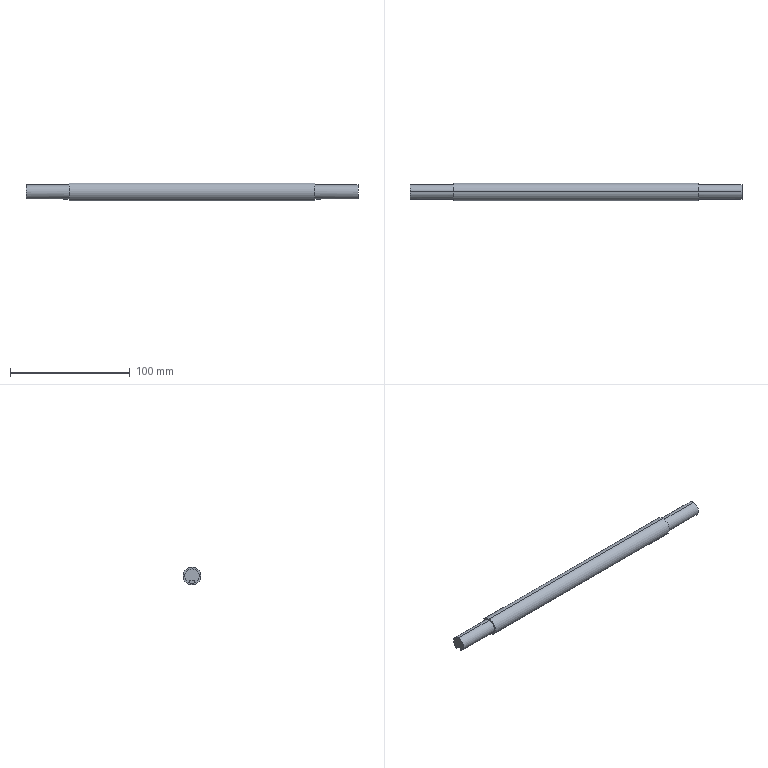Component | SolidWorks | ReducerCoupling-1 | 1 solid | 18 faces | box 277 x 15 x 15 mm | volume 43778 mm3 | plane 12 | cylinder 6 | commonest cylinder face diameters 12 x4 15 x2
build123d program:
from build123d import *

# Parameters (mm, degrees)
SKETCH2_W      = 4
SKETCH2_H      = 3.974
EXTRUDE1_DEPTH = 31
SKETCH3_W      = 4
SKETCH3_H      = 4.547
EXTRUDE2_DEPTH = 31


with BuildPart() as part:
    # Sketch1 → Revolve1 (revolve)
    with BuildSketch(Plane.XY, mode=Mode.PRIVATE) as revolve1_sk:
        Polygon((0, 106.041), (6, 106.041), (6, 70.041), (7.5, 70.041), (7.5, -134.959), (6, -134.959), (6, -170.959), (0, -170.959), align=None)
    revolve(revolve1_sk.sketch.rotate(Axis((0, 0, 0), (0, 1, 0)), 90), axis=Axis((0, 0, 0), (0, 1, 0)))

    # Sketch2 → Extrude1 (cut)
    with BuildSketch(Plane(origin=(0, 106.041, 0), x_dir=(1, 0, 0), z_dir=(0, 1, 0))):
        with Locations((0, 5.487)):
            Rectangle(SKETCH2_W, SKETCH2_H)
    extrude(amount=-EXTRUDE1_DEPTH, mode=Mode.SUBTRACT)

    # Sketch3 → Extrude2 (cut)
    with BuildSketch(Plane.XZ.offset(170.959)):
        with Locations((0, -5.774)):
            Rectangle(SKETCH3_W, SKETCH3_H)
    extrude(amount=-EXTRUDE2_DEPTH, mode=Mode.SUBTRACT)


solid = part.part

# Placed as in the assembly
solid = solid.moved(Location((52.758, 175.983, 58.736), (0, 0, 90)))
STEP:
#1=COLOUR_RGB('',0.7922,0.8196,0.9333);
#2=FILL_AREA_STYLE_COLOUR('',#1);
#3=FILL_AREA_STYLE('',(#2));
#4=SURFACE_STYLE_FILL_AREA(#3);
#5=SURFACE_SIDE_STYLE('',(#4));
#6=SURFACE_STYLE_USAGE(.BOTH.,#5);
#7=PRESENTATION_STYLE_ASSIGNMENT((#6));
#8=CARTESIAN_POINT('',(7.39,6.928,2.076));
#9=VERTEX_POINT('',#8);
#10=CARTESIAN_POINT('',(7.39,6.928,2.549));
#11=VERTEX_POINT('',#10);
#12=CARTESIAN_POINT('',(7.39,6.928,2.312));
#13=DIRECTION('',(1.,0.,0.));
#14=DIRECTION('',(0.,0.,-1.));
#15=AXIS2_PLACEMENT_3D('',#12,#13,#14);
#16=CIRCLE('',#15,0.2362);
#17=EDGE_CURVE('',#9,#11,#16,.T.);
#18=ORIENTED_EDGE('',*,*,#17,.T.);
#19=CARTESIAN_POINT('',(8.808,6.928,2.549));
#20=VERTEX_POINT('',#19);
#21=CARTESIAN_POINT('',(2.077,6.928,2.549));
#22=DIRECTION('',(1.,0.,0.));
#23=VECTOR('',#22,39.37);
#24=LINE('',#21,#23);
#25=EDGE_CURVE('',#11,#20,#24,.T.);
#26=ORIENTED_EDGE('',*,*,#25,.T.);
#27=CARTESIAN_POINT('',(8.808,7.007,2.09));
#28=VERTEX_POINT('',#27);
#29=CARTESIAN_POINT('',(8.808,6.928,2.312));
#30=DIRECTION('',(1.,0.,0.));
#31=DIRECTION('',(0.,0.,-1.));
#32=AXIS2_PLACEMENT_3D('',#29,#30,#31);
#33=CIRCLE('',#32,0.2362);
#34=EDGE_CURVE('',#28,#20,#33,.T.);
#35=ORIENTED_EDGE('',*,*,#34,.F.);
#36=CARTESIAN_POINT('',(7.587,7.007,2.09));
#37=VERTEX_POINT('',#36);
#38=CARTESIAN_POINT('',(2.077,7.007,2.09));
#39=DIRECTION('',(1.,0.,0.));
#40=VECTOR('',#39,39.37);
#41=LINE('',#38,#40);
#42=EDGE_CURVE('',#37,#28,#41,.T.);
#43=ORIENTED_EDGE('',*,*,#42,.F.);
#44=CARTESIAN_POINT('',(7.587,6.928,2.076));
#45=VERTEX_POINT('',#44);
#46=CARTESIAN_POINT('',(7.587,6.928,2.312));
#47=DIRECTION('',(-1.,-0.,-0.));
#48=DIRECTION('',(0.,-0.,-1.));
#49=AXIS2_PLACEMENT_3D('',#46,#47,#48);
#50=CIRCLE('',#49,0.2362);
#51=EDGE_CURVE('',#37,#45,#50,.T.);
#52=ORIENTED_EDGE('',*,*,#51,.T.);
#53=CARTESIAN_POINT('',(2.077,6.928,2.076));
#54=DIRECTION('',(1.,0.,0.));
#55=VECTOR('',#54,39.37);
#56=LINE('',#53,#55);
#57=EDGE_CURVE('',#9,#45,#56,.T.);
#58=ORIENTED_EDGE('',*,*,#57,.F.);
#59=EDGE_LOOP('',(#18,#26,#35,#43,#52,#58));
#60=FACE_OUTER_BOUND('',#59,.T.);
#61=CARTESIAN_POINT('',(2.077,6.928,2.312));
#62=DIRECTION('',(1.,0.,0.));
#63=DIRECTION('',(0.,0.,-1.));
#64=AXIS2_PLACEMENT_3D('',#61,#62,#63);
#65=CYLINDRICAL_SURFACE('',#64,0.2362);
#66=ADVANCED_FACE('',(#60),#65,.T.);
#67=CARTESIAN_POINT('',(-0.6805,6.928,2.017));
#68=VERTEX_POINT('',#67);
#69=CARTESIAN_POINT('',(-0.6805,6.928,2.608));
#70=VERTEX_POINT('',#69);
#71=CARTESIAN_POINT('',(-0.6805,6.928,2.312));
#72=DIRECTION('',(1.,0.,0.));
#73=DIRECTION('',(0.,0.,-1.));
#74=AXIS2_PLACEMENT_3D('',#71,#72,#73);
#75=CIRCLE('',#74,0.2953);
#76=EDGE_CURVE('',#68,#70,#75,.T.);
#77=ORIENTED_EDGE('',*,*,#76,.T.);
#78=CARTESIAN_POINT('',(7.39,6.928,2.608));
#79=VERTEX_POINT('',#78);
#80=CARTESIAN_POINT('',(2.077,6.928,2.608));
#81=DIRECTION('',(1.,0.,0.));
#82=VECTOR('',#81,39.37);
#83=LINE('',#80,#82);
#84=EDGE_CURVE('',#70,#79,#83,.T.);
#85=ORIENTED_EDGE('',*,*,#84,.T.);
#86=CARTESIAN_POINT('',(7.39,6.928,2.017));
#87=VERTEX_POINT('',#86);
#88=CARTESIAN_POINT('',(7.39,6.928,2.312));
#89=DIRECTION('',(1.,0.,0.));
#90=DIRECTION('',(0.,0.,-1.));
#91=AXIS2_PLACEMENT_3D('',#88,#89,#90);
#92=CIRCLE('',#91,0.2953);
#93=EDGE_CURVE('',#87,#79,#92,.T.);
#94=ORIENTED_EDGE('',*,*,#93,.F.);
#95=CARTESIAN_POINT('',(2.077,6.928,2.017));
#96=DIRECTION('',(1.,0.,0.));
#97=VECTOR('',#96,39.37);
#98=LINE('',#95,#97);
#99=EDGE_CURVE('',#68,#87,#98,.T.);
#100=ORIENTED_EDGE('',*,*,#99,.F.);
#101=EDGE_LOOP('',(#77,#85,#94,#100));
#102=FACE_OUTER_BOUND('',#101,.T.);
#103=CARTESIAN_POINT('',(2.077,6.928,2.312));
#104=DIRECTION('',(1.,0.,0.));
#105=DIRECTION('',(0.,0.,-1.));
#106=AXIS2_PLACEMENT_3D('',#103,#104,#105);
#107=CYLINDRICAL_SURFACE('',#106,0.2953);
#108=ADVANCED_FACE('',(#102),#107,.T.);
#109=CARTESIAN_POINT('',(-2.098,7.007,2.09));
#110=VERTEX_POINT('',#109);
#111=CARTESIAN_POINT('',(-2.098,6.928,2.549));
#112=VERTEX_POINT('',#111);
#113=CARTESIAN_POINT('',(-2.098,6.928,2.312));
#114=DIRECTION('',(1.,0.,0.));
#115=DIRECTION('',(0.,0.,-1.));
#116=AXIS2_PLACEMENT_3D('',#113,#114,#115);
#117=CIRCLE('',#116,0.2362);
#118=EDGE_CURVE('',#110,#112,#117,.T.);
#119=ORIENTED_EDGE('',*,*,#118,.T.);
#120=CARTESIAN_POINT('',(-0.6805,6.928,2.549));
#121=VERTEX_POINT('',#120);
#122=CARTESIAN_POINT('',(2.077,6.928,2.549));
#123=DIRECTION('',(1.,0.,0.));
#124=VECTOR('',#123,39.37);
#125=LINE('',#122,#124);
#126=EDGE_CURVE('',#112,#121,#125,.T.);
#127=ORIENTED_EDGE('',*,*,#126,.T.);
#128=CARTESIAN_POINT('',(-0.6805,6.928,2.076));
#129=VERTEX_POINT('',#128);
#130=CARTESIAN_POINT('',(-0.6805,6.928,2.312));
#131=DIRECTION('',(1.,0.,0.));
#132=DIRECTION('',(0.,0.,-1.));
#133=AXIS2_PLACEMENT_3D('',#130,#131,#132);
#134=CIRCLE('',#133,0.2362);
#135=EDGE_CURVE('',#129,#121,#134,.T.);
#136=ORIENTED_EDGE('',*,*,#135,.F.);
#137=CARTESIAN_POINT('',(-0.8773,6.928,2.076));
#138=VERTEX_POINT('',#137);
#139=CARTESIAN_POINT('',(2.077,6.928,2.076));
#140=DIRECTION('',(1.,0.,0.));
#141=VECTOR('',#140,39.37);
#142=LINE('',#139,#141);
#143=EDGE_CURVE('',#138,#129,#142,.T.);
#144=ORIENTED_EDGE('',*,*,#143,.F.);
#145=CARTESIAN_POINT('',(-0.8773,7.007,2.09));
#146=VERTEX_POINT('',#145);
#147=CARTESIAN_POINT('',(-0.8773,6.928,2.312));
#148=DIRECTION('',(1.,0.,0.));
#149=DIRECTION('',(0.,0.,1.));
#150=AXIS2_PLACEMENT_3D('',#147,#148,#149);
#151=CIRCLE('',#150,0.2362);
#152=EDGE_CURVE('',#138,#146,#151,.T.);
#153=ORIENTED_EDGE('',*,*,#152,.T.);
#154=CARTESIAN_POINT('',(2.077,7.007,2.09));
#155=DIRECTION('',(1.,0.,0.));
#156=VECTOR('',#155,39.37);
#157=LINE('',#154,#156);
#158=EDGE_CURVE('',#110,#146,#157,.T.);
#159=ORIENTED_EDGE('',*,*,#158,.F.);
#160=EDGE_LOOP('',(#119,#127,#136,#144,#153,#159));
#161=FACE_OUTER_BOUND('',#160,.T.);
#162=CARTESIAN_POINT('',(2.077,6.928,2.312));
#163=DIRECTION('',(1.,0.,0.));
#164=DIRECTION('',(0.,0.,-1.));
#165=AXIS2_PLACEMENT_3D('',#162,#163,#164);
#166=CYLINDRICAL_SURFACE('',#165,0.2362);
#167=ADVANCED_FACE('',(#161),#166,.T.);
#168=CARTESIAN_POINT('',(-2.098,6.85,2.09));
#169=VERTEX_POINT('',#168);
#170=CARTESIAN_POINT('',(-2.098,6.85,2.175));
#171=VERTEX_POINT('',#170);
#172=CARTESIAN_POINT('',(-2.098,6.85,2.018));
#173=DIRECTION('',(-0.,0.,1.));
#174=VECTOR('',#173,39.37);
#175=LINE('',#172,#174);
#176=EDGE_CURVE('',#169,#171,#175,.T.);
#177=ORIENTED_EDGE('',*,*,#176,.F.);
#178=CARTESIAN_POINT('',(-2.098,6.928,2.312));
#179=DIRECTION('',(1.,0.,0.));
#180=DIRECTION('',(0.,0.,-1.));
#181=AXIS2_PLACEMENT_3D('',#178,#179,#180);
#182=CIRCLE('',#181,0.2362);
#183=EDGE_CURVE('',#112,#169,#182,.T.);
#184=ORIENTED_EDGE('',*,*,#183,.F.);
#185=ORIENTED_EDGE('',*,*,#118,.F.);
#186=CARTESIAN_POINT('',(-2.098,7.007,2.175));
#187=VERTEX_POINT('',#186);
#188=CARTESIAN_POINT('',(-2.098,7.007,2.018));
#189=DIRECTION('',(0.,0.,-1.));
#190=VECTOR('',#189,39.37);
#191=LINE('',#188,#190);
#192=EDGE_CURVE('',#187,#110,#191,.T.);
#193=ORIENTED_EDGE('',*,*,#192,.F.);
#194=CARTESIAN_POINT('',(-2.098,6.85,2.175));
#195=DIRECTION('',(-0.,1.,-0.));
#196=VECTOR('',#195,39.37);
#197=LINE('',#194,#196);
#198=EDGE_CURVE('',#171,#187,#197,.T.);
#199=ORIENTED_EDGE('',*,*,#198,.F.);
#200=EDGE_LOOP('',(#177,#184,#185,#193,#199));
#201=FACE_OUTER_BOUND('',#200,.T.);
#202=CARTESIAN_POINT('',(-2.098,6.928,2.312));
#203=DIRECTION('',(-1.,-0.,-0.));
#204=DIRECTION('',(-0.,0.,1.));
#205=AXIS2_PLACEMENT_3D('',#202,#203,#204);
#206=PLANE('',#205);
#207=ADVANCED_FACE('',(#201),#206,.T.);
#208=ORIENTED_EDGE('',*,*,#126,.F.);
#209=ORIENTED_EDGE('',*,*,#183,.T.);
#210=CARTESIAN_POINT('',(-0.8773,6.85,2.09));
#211=VERTEX_POINT('',#210);
#212=CARTESIAN_POINT('',(2.077,6.85,2.09));
#213=DIRECTION('',(-1.,-0.,-0.));
#214=VECTOR('',#213,39.37);
#215=LINE('',#212,#214);
#216=EDGE_CURVE('',#211,#169,#215,.T.);
#217=ORIENTED_EDGE('',*,*,#216,.F.);
#218=CARTESIAN_POINT('',(-0.8773,6.928,2.312));
#219=DIRECTION('',(1.,0.,0.));
#220=DIRECTION('',(0.,0.,1.));
#221=AXIS2_PLACEMENT_3D('',#218,#219,#220);
#222=CIRCLE('',#221,0.2362);
#223=EDGE_CURVE('',#211,#138,#222,.T.);
#224=ORIENTED_EDGE('',*,*,#223,.T.);
#225=ORIENTED_EDGE('',*,*,#143,.T.);
#226=CARTESIAN_POINT('',(-0.6805,6.928,2.312));
#227=DIRECTION('',(1.,0.,0.));
#228=DIRECTION('',(0.,0.,-1.));
#229=AXIS2_PLACEMENT_3D('',#226,#227,#228);
#230=CIRCLE('',#229,0.2362);
#231=EDGE_CURVE('',#121,#129,#230,.T.);
#232=ORIENTED_EDGE('',*,*,#231,.F.);
#233=EDGE_LOOP('',(#208,#209,#217,#224,#225,#232));
#234=FACE_OUTER_BOUND('',#233,.T.);
#235=CARTESIAN_POINT('',(2.077,6.928,2.312));
#236=DIRECTION('',(1.,0.,0.));
#237=DIRECTION('',(0.,0.,-1.));
#238=AXIS2_PLACEMENT_3D('',#235,#236,#237);
#239=CYLINDRICAL_SURFACE('',#238,0.2362);
#240=ADVANCED_FACE('',(#234),#239,.T.);
#241=ORIENTED_EDGE('',*,*,#135,.T.);
#242=ORIENTED_EDGE('',*,*,#231,.T.);
#243=EDGE_LOOP('',(#241,#242));
#244=FACE_BOUND('',#243,.T.);
#245=ORIENTED_EDGE('',*,*,#76,.F.);
#246=CARTESIAN_POINT('',(-0.6805,6.928,2.312));
#247=DIRECTION('',(1.,0.,0.));
#248=DIRECTION('',(0.,0.,-1.));
#249=AXIS2_PLACEMENT_3D('',#246,#247,#248);
#250=CIRCLE('',#249,0.2953);
#251=EDGE_CURVE('',#70,#68,#250,.T.);
#252=ORIENTED_EDGE('',*,*,#251,.F.);
#253=EDGE_LOOP('',(#245,#252));
#254=FACE_OUTER_BOUND('',#253,.T.);
#255=CARTESIAN_POINT('',(-0.6805,7.165,2.312));
#256=DIRECTION('',(-1.,-0.,-0.));
#257=DIRECTION('',(-0.,0.,1.));
#258=AXIS2_PLACEMENT_3D('',#255,#256,#257);
#259=PLANE('',#258);
#260=ADVANCED_FACE('',(#244,#254),#259,.T.);
#261=ORIENTED_EDGE('',*,*,#84,.F.);
#262=ORIENTED_EDGE('',*,*,#251,.T.);
#263=ORIENTED_EDGE('',*,*,#99,.T.);
#264=CARTESIAN_POINT('',(7.39,6.928,2.312));
#265=DIRECTION('',(1.,0.,0.));
#266=DIRECTION('',(0.,0.,-1.));
#267=AXIS2_PLACEMENT_3D('',#264,#265,#266);
#268=CIRCLE('',#267,0.2953);
#269=EDGE_CURVE('',#79,#87,#268,.T.);
#270=ORIENTED_EDGE('',*,*,#269,.F.);
#271=EDGE_LOOP('',(#261,#262,#263,#270));
#272=FACE_OUTER_BOUND('',#271,.T.);
#273=CARTESIAN_POINT('',(2.077,6.928,2.312));
#274=DIRECTION('',(1.,0.,0.));
#275=DIRECTION('',(0.,0.,-1.));
#276=AXIS2_PLACEMENT_3D('',#273,#274,#275);
#277=CYLINDRICAL_SURFACE('',#276,0.2953);
#278=ADVANCED_FACE('',(#272),#277,.T.);
#279=ORIENTED_EDGE('',*,*,#93,.T.);
#280=ORIENTED_EDGE('',*,*,#269,.T.);
#281=EDGE_LOOP('',(#279,#280));
#282=FACE_OUTER_BOUND('',#281,.T.);
#283=ORIENTED_EDGE('',*,*,#17,.F.);
#284=CARTESIAN_POINT('',(7.39,6.928,2.312));
#285=DIRECTION('',(1.,0.,0.));
#286=DIRECTION('',(0.,0.,-1.));
#287=AXIS2_PLACEMENT_3D('',#284,#285,#286);
#288=CIRCLE('',#287,0.2362);
#289=EDGE_CURVE('',#11,#9,#288,.T.);
#290=ORIENTED_EDGE('',*,*,#289,.F.);
#291=EDGE_LOOP('',(#283,#290));
#292=FACE_BOUND('',#291,.T.);
#293=CARTESIAN_POINT('',(7.39,7.224,2.312));
#294=DIRECTION('',(1.,0.,0.));
#295=DIRECTION('',(0.,-0.,-1.));
#296=AXIS2_PLACEMENT_3D('',#293,#294,#295);
#297=PLANE('',#296);
#298=ADVANCED_FACE('',(#282,#292),#297,.T.);
#299=ORIENTED_EDGE('',*,*,#25,.F.);
#300=ORIENTED_EDGE('',*,*,#289,.T.);
#301=ORIENTED_EDGE('',*,*,#57,.T.);
#302=CARTESIAN_POINT('',(7.587,6.85,2.09));
#303=VERTEX_POINT('',#302);
#304=CARTESIAN_POINT('',(7.587,6.928,2.312));
#305=DIRECTION('',(-1.,-0.,-0.));
#306=DIRECTION('',(0.,0.,-1.));
#307=AXIS2_PLACEMENT_3D('',#304,#305,#306);
#308=CIRCLE('',#307,0.2362);
#309=EDGE_CURVE('',#45,#303,#308,.T.);
#310=ORIENTED_EDGE('',*,*,#309,.T.);
#311=CARTESIAN_POINT('',(8.808,6.85,2.09));
#312=VERTEX_POINT('',#311);
#313=CARTESIAN_POINT('',(2.077,6.85,2.09));
#314=DIRECTION('',(-1.,-0.,-0.));
#315=VECTOR('',#314,39.37);
#316=LINE('',#313,#315);
#317=EDGE_CURVE('',#312,#303,#316,.T.);
#318=ORIENTED_EDGE('',*,*,#317,.F.);
#319=CARTESIAN_POINT('',(8.808,6.928,2.312));
#320=DIRECTION('',(1.,0.,0.));
#321=DIRECTION('',(0.,0.,-1.));
#322=AXIS2_PLACEMENT_3D('',#319,#320,#321);
#323=CIRCLE('',#322,0.2362);
#324=EDGE_CURVE('',#20,#312,#323,.T.);
#325=ORIENTED_EDGE('',*,*,#324,.F.);
#326=EDGE_LOOP('',(#299,#300,#301,#310,#318,#325));
#327=FACE_OUTER_BOUND('',#326,.T.);
#328=CARTESIAN_POINT('',(2.077,6.928,2.312));
#329=DIRECTION('',(1.,0.,0.));
#330=DIRECTION('',(0.,0.,-1.));
#331=AXIS2_PLACEMENT_3D('',#328,#329,#330);
#332=CYLINDRICAL_SURFACE('',#331,0.2362);
#333=ADVANCED_FACE('',(#327),#332,.T.);
#334=CARTESIAN_POINT('',(8.808,6.85,2.175));
#335=VERTEX_POINT('',#334);
#336=CARTESIAN_POINT('',(8.808,6.85,2.175));
#337=DIRECTION('',(0.,-0.,-1.));
#338=VECTOR('',#337,39.37);
#339=LINE('',#336,#338);
#340=EDGE_CURVE('',#335,#312,#339,.T.);
#341=ORIENTED_EDGE('',*,*,#340,.F.);
#342=CARTESIAN_POINT('',(8.808,7.007,2.175));
#343=VERTEX_POINT('',#342);
#344=CARTESIAN_POINT('',(8.808,6.85,2.175));
#345=DIRECTION('',(0.,-1.,0.));
#346=VECTOR('',#345,39.37);
#347=LINE('',#344,#346);
#348=EDGE_CURVE('',#343,#335,#347,.T.);
#349=ORIENTED_EDGE('',*,*,#348,.F.);
#350=CARTESIAN_POINT('',(8.808,7.007,2.312));
#351=DIRECTION('',(-0.,0.,1.));
#352=VECTOR('',#351,39.37);
#353=LINE('',#350,#352);
#354=EDGE_CURVE('',#28,#343,#353,.T.);
#355=ORIENTED_EDGE('',*,*,#354,.F.);
#356=ORIENTED_EDGE('',*,*,#34,.T.);
#357=ORIENTED_EDGE('',*,*,#324,.T.);
#358=EDGE_LOOP('',(#341,#349,#355,#356,#357));
#359=FACE_OUTER_BOUND('',#358,.T.);
#360=CARTESIAN_POINT('',(8.808,7.165,2.312));
#361=DIRECTION('',(1.,0.,0.));
#362=DIRECTION('',(0.,-0.,-1.));
#363=AXIS2_PLACEMENT_3D('',#360,#361,#362);
#364=PLANE('',#363);
#365=ADVANCED_FACE('',(#359),#364,.T.);
#366=ORIENTED_EDGE('',*,*,#216,.T.);
#367=ORIENTED_EDGE('',*,*,#176,.T.);
#368=CARTESIAN_POINT('',(-0.8773,6.85,2.175));
#369=VERTEX_POINT('',#368);
#370=CARTESIAN_POINT('',(-0.8773,6.85,2.175));
#371=DIRECTION('',(-1.,-0.,-0.));
#372=VECTOR('',#371,39.37);
#373=LINE('',#370,#372);
#374=EDGE_CURVE('',#369,#171,#373,.T.);
#375=ORIENTED_EDGE('',*,*,#374,.F.);
#376=CARTESIAN_POINT('',(-0.8773,6.85,2.018));
#377=DIRECTION('',(-0.,0.,1.));
#378=VECTOR('',#377,39.37);
#379=LINE('',#376,#378);
#380=EDGE_CURVE('',#211,#369,#379,.T.);
#381=ORIENTED_EDGE('',*,*,#380,.F.);
#382=EDGE_LOOP('',(#366,#367,#375,#381));
#383=FACE_OUTER_BOUND('',#382,.T.);
#384=CARTESIAN_POINT('',(-0.8773,6.85,2.018));
#385=DIRECTION('',(0.,-1.,0.));
#386=DIRECTION('',(-0.,0.,1.));
#387=AXIS2_PLACEMENT_3D('',#384,#385,#386);
#388=PLANE('',#387);
#389=ADVANCED_FACE('',(#383),#388,.F.);
#390=ORIENTED_EDGE('',*,*,#158,.T.);
#391=CARTESIAN_POINT('',(-0.8773,7.007,2.175));
#392=VERTEX_POINT('',#391);
#393=CARTESIAN_POINT('',(-0.8773,7.007,2.018));
#394=DIRECTION('',(0.,0.,-1.));
#395=VECTOR('',#394,39.37);
#396=LINE('',#393,#395);
#397=EDGE_CURVE('',#392,#146,#396,.T.);
#398=ORIENTED_EDGE('',*,*,#397,.F.);
#399=CARTESIAN_POINT('',(-0.8773,7.007,2.175));
#400=DIRECTION('',(-1.,-0.,-0.));
#401=VECTOR('',#400,39.37);
#402=LINE('',#399,#401);
#403=EDGE_CURVE('',#392,#187,#402,.T.);
#404=ORIENTED_EDGE('',*,*,#403,.T.);
#405=ORIENTED_EDGE('',*,*,#192,.T.);
#406=EDGE_LOOP('',(#390,#398,#404,#405));
#407=FACE_OUTER_BOUND('',#406,.T.);
#408=CARTESIAN_POINT('',(-0.8773,7.007,2.018));
#409=DIRECTION('',(-0.,1.,0.));
#410=DIRECTION('',(0.,0.,-1.));
#411=AXIS2_PLACEMENT_3D('',#408,#409,#410);
#412=PLANE('',#411);
#413=ADVANCED_FACE('',(#407),#412,.F.);
#414=ORIENTED_EDGE('',*,*,#198,.T.);
#415=ORIENTED_EDGE('',*,*,#403,.F.);
#416=CARTESIAN_POINT('',(-0.8773,6.85,2.175));
#417=DIRECTION('',(-0.,1.,-0.));
#418=VECTOR('',#417,39.37);
#419=LINE('',#416,#418);
#420=EDGE_CURVE('',#369,#392,#419,.T.);
#421=ORIENTED_EDGE('',*,*,#420,.F.);
#422=ORIENTED_EDGE('',*,*,#374,.T.);
#423=EDGE_LOOP('',(#414,#415,#421,#422));
#424=FACE_OUTER_BOUND('',#423,.T.);
#425=CARTESIAN_POINT('',(-0.8773,6.85,2.175));
#426=DIRECTION('',(-0.,0.,1.));
#427=DIRECTION('',(-0.,1.,-0.));
#428=AXIS2_PLACEMENT_3D('',#425,#426,#427);
#429=PLANE('',#428);
#430=ADVANCED_FACE('',(#424),#429,.F.);
#431=ORIENTED_EDGE('',*,*,#380,.T.);
#432=ORIENTED_EDGE('',*,*,#420,.T.);
#433=ORIENTED_EDGE('',*,*,#397,.T.);
#434=ORIENTED_EDGE('',*,*,#152,.F.);
#435=ORIENTED_EDGE('',*,*,#223,.F.);
#436=EDGE_LOOP('',(#431,#432,#433,#434,#435));
#437=FACE_OUTER_BOUND('',#436,.T.);
#438=CARTESIAN_POINT('',(-0.8773,6.85,2.175));
#439=DIRECTION('',(-1.,-0.,-0.));
#440=DIRECTION('',(-0.,0.,1.));
#441=AXIS2_PLACEMENT_3D('',#438,#439,#440);
#442=PLANE('',#441);
#443=ADVANCED_FACE('',(#437),#442,.T.);
#444=ORIENTED_EDGE('',*,*,#317,.T.);
#445=CARTESIAN_POINT('',(7.587,6.85,2.175));
#446=VERTEX_POINT('',#445);
#447=CARTESIAN_POINT('',(7.587,6.85,2.175));
#448=DIRECTION('',(0.,-0.,-1.));
#449=VECTOR('',#448,39.37);
#450=LINE('',#447,#449);
#451=EDGE_CURVE('',#446,#303,#450,.T.);
#452=ORIENTED_EDGE('',*,*,#451,.F.);
#453=CARTESIAN_POINT('',(7.587,6.85,2.175));
#454=DIRECTION('',(1.,0.,0.));
#455=VECTOR('',#454,39.37);
#456=LINE('',#453,#455);
#457=EDGE_CURVE('',#446,#335,#456,.T.);
#458=ORIENTED_EDGE('',*,*,#457,.T.);
#459=ORIENTED_EDGE('',*,*,#340,.T.);
#460=EDGE_LOOP('',(#444,#452,#458,#459));
#461=FACE_OUTER_BOUND('',#460,.T.);
#462=CARTESIAN_POINT('',(7.587,6.85,2.175));
#463=DIRECTION('',(0.,-1.,0.));
#464=DIRECTION('',(-0.,0.,1.));
#465=AXIS2_PLACEMENT_3D('',#462,#463,#464);
#466=PLANE('',#465);
#467=ADVANCED_FACE('',(#461),#466,.F.);
#468=ORIENTED_EDGE('',*,*,#348,.T.);
#469=ORIENTED_EDGE('',*,*,#457,.F.);
#470=CARTESIAN_POINT('',(7.587,7.007,2.175));
#471=VERTEX_POINT('',#470);
#472=CARTESIAN_POINT('',(7.587,6.85,2.175));
#473=DIRECTION('',(0.,-1.,0.));
#474=VECTOR('',#473,39.37);
#475=LINE('',#472,#474);
#476=EDGE_CURVE('',#471,#446,#475,.T.);
#477=ORIENTED_EDGE('',*,*,#476,.F.);
#478=CARTESIAN_POINT('',(7.587,7.007,2.175));
#479=DIRECTION('',(1.,0.,0.));
#480=VECTOR('',#479,39.37);
#481=LINE('',#478,#480);
#482=EDGE_CURVE('',#471,#343,#481,.T.);
#483=ORIENTED_EDGE('',*,*,#482,.T.);
#484=EDGE_LOOP('',(#468,#469,#477,#483));
#485=FACE_OUTER_BOUND('',#484,.T.);
#486=CARTESIAN_POINT('',(7.587,6.85,2.175));
#487=DIRECTION('',(-0.,0.,1.));
#488=DIRECTION('',(-0.,1.,-0.));
#489=AXIS2_PLACEMENT_3D('',#486,#487,#488);
#490=PLANE('',#489);
#491=ADVANCED_FACE('',(#485),#490,.F.);
#492=ORIENTED_EDGE('',*,*,#42,.T.);
#493=ORIENTED_EDGE('',*,*,#354,.T.);
#494=ORIENTED_EDGE('',*,*,#482,.F.);
#495=CARTESIAN_POINT('',(7.587,7.007,2.175));
#496=DIRECTION('',(-0.,0.,1.));
#497=VECTOR('',#496,39.37);
#498=LINE('',#495,#497);
#499=EDGE_CURVE('',#37,#471,#498,.T.);
#500=ORIENTED_EDGE('',*,*,#499,.F.);
#501=EDGE_LOOP('',(#492,#493,#494,#500));
#502=FACE_OUTER_BOUND('',#501,.T.);
#503=CARTESIAN_POINT('',(7.587,7.007,2.175));
#504=DIRECTION('',(-0.,1.,-0.));
#505=DIRECTION('',(0.,-0.,-1.));
#506=AXIS2_PLACEMENT_3D('',#503,#504,#505);
#507=PLANE('',#506);
#508=ADVANCED_FACE('',(#502),#507,.F.);
#509=ORIENTED_EDGE('',*,*,#499,.T.);
#510=ORIENTED_EDGE('',*,*,#476,.T.);
#511=ORIENTED_EDGE('',*,*,#451,.T.);
#512=ORIENTED_EDGE('',*,*,#309,.F.);
#513=ORIENTED_EDGE('',*,*,#51,.F.);
#514=EDGE_LOOP('',(#509,#510,#511,#512,#513));
#515=FACE_OUTER_BOUND('',#514,.T.);
#516=CARTESIAN_POINT('',(7.587,6.85,1.996));
#517=DIRECTION('',(1.,0.,0.));
#518=DIRECTION('',(0.,-0.,-1.));
#519=AXIS2_PLACEMENT_3D('',#516,#517,#518);
#520=PLANE('',#519);
#521=ADVANCED_FACE('',(#515),#520,.T.);
#522=CLOSED_SHELL('',(#66,#108,#167,#207,#240,#260,#278,#298,#333,#365,#389,#413,#430,#443,#467,#491,#508,#521));
#523=MANIFOLD_SOLID_BREP('',#522);
#524=STYLED_ITEM('',(#7),#523);
#525=(LENGTH_UNIT()NAMED_UNIT(*)SI_UNIT($,.METRE.));
#526=LENGTH_MEASURE_WITH_UNIT(LENGTH_MEASURE(0.0254),#525);
#527=DIMENSIONAL_EXPONENTS(1.,0.,0.,0.,0.,0.,0.);
#528=(CONVERSION_BASED_UNIT('',#526)LENGTH_UNIT()NAMED_UNIT(#527));
#529=UNCERTAINTY_MEASURE_WITH_UNIT(LENGTH_MEASURE(0.00001),#528,'','');
#530=(NAMED_UNIT(*)PLANE_ANGLE_UNIT()SI_UNIT($,.RADIAN.));
#531=(NAMED_UNIT(*)SI_UNIT($,.STERADIAN.)SOLID_ANGLE_UNIT());
#532=(GEOMETRIC_REPRESENTATION_CONTEXT(3)GLOBAL_UNCERTAINTY_ASSIGNED_CONTEXT((#529))GLOBAL_UNIT_ASSIGNED_CONTEXT((#528,#530,#531))REPRESENTATION_CONTEXT('',''));
#533=MECHANICAL_DESIGN_GEOMETRIC_PRESENTATION_REPRESENTATION('',(#524),#532);
#534=CARTESIAN_POINT('',(0.,0.,0.));
#535=DIRECTION('',(0.,0.,1.));
#536=DIRECTION('',(1.,0.,0.));
#537=AXIS2_PLACEMENT_3D('',#534,#535,#536);
#538=(LENGTH_UNIT()NAMED_UNIT(*)SI_UNIT($,.METRE.));
#539=LENGTH_MEASURE_WITH_UNIT(LENGTH_MEASURE(0.0254),#538);
#540=DIMENSIONAL_EXPONENTS(1.,0.,0.,0.,0.,0.,0.);
#541=(CONVERSION_BASED_UNIT('',#539)LENGTH_UNIT()NAMED_UNIT(#540));
#542=UNCERTAINTY_MEASURE_WITH_UNIT(LENGTH_MEASURE(0.00001),#541,'','');
#543=(NAMED_UNIT(*)PLANE_ANGLE_UNIT()SI_UNIT($,.RADIAN.));
#544=(NAMED_UNIT(*)SI_UNIT($,.STERADIAN.)SOLID_ANGLE_UNIT());
#545=(GEOMETRIC_REPRESENTATION_CONTEXT(3)GLOBAL_UNCERTAINTY_ASSIGNED_CONTEXT((#542))GLOBAL_UNIT_ASSIGNED_CONTEXT((#541,#543,#544))REPRESENTATION_CONTEXT('',''));
#546=ADVANCED_BREP_SHAPE_REPRESENTATION('',(#523,#537),#545);
#547=PRESENTATION_LAYER_ASSIGNMENT('','',(#524));